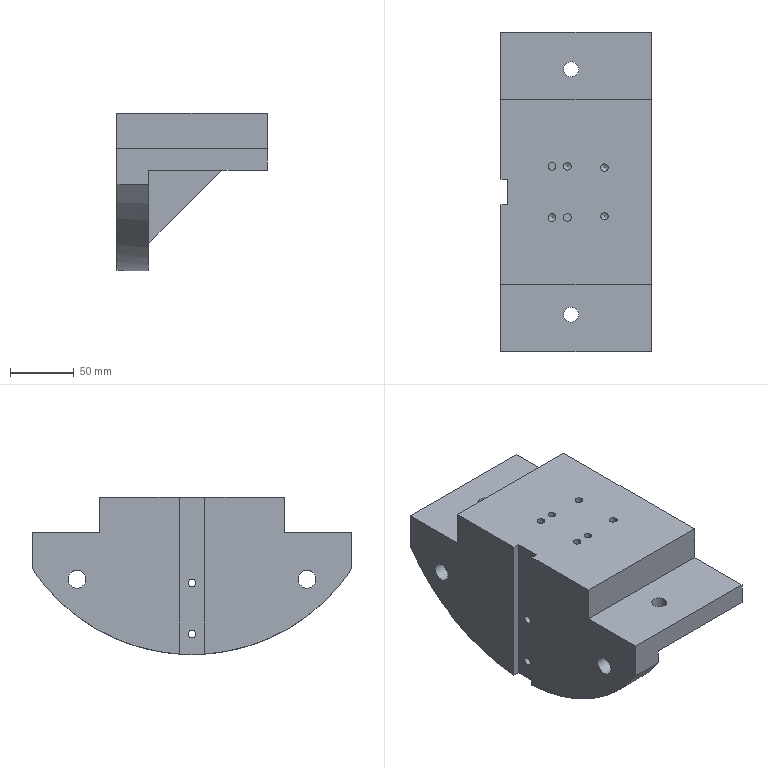Component | NX | ANGLE_BAR | 1 solid | 40 faces | volume 1346280 mm3 | plane 23 | cylinder 13 | cone 4 | commonest cylinder face diameters 6 x8 14 x2 12 x2 300 x1